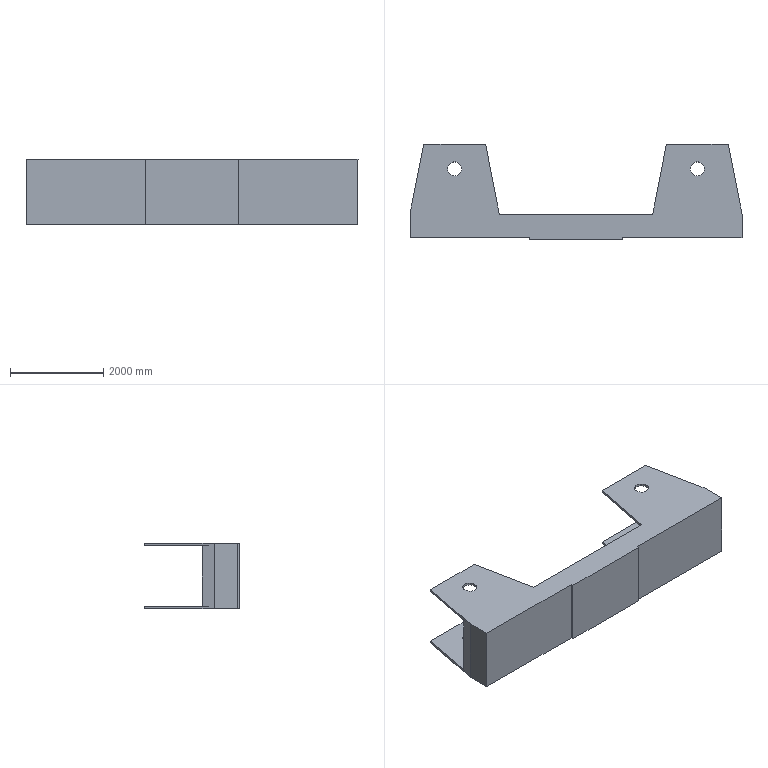Component | SolidWorks | RunningMechanism-4_Part13-1 | 1 solid | 40 faces | volume 1594643558 mm3 | plane 32 | cylinder 8 | commonest cylinder face diameters 300 x8